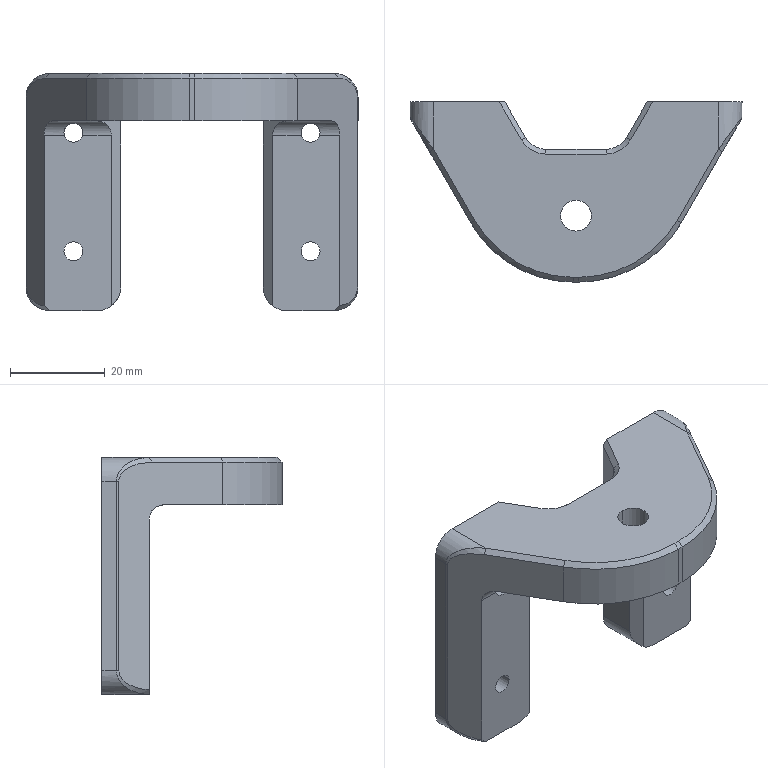Component | SolidWorks | DZ.KX.203-TC1505-30-09-01-05-28-2 | 1 solid | 68 faces | volume 29569 mm3 | plane 31 | cylinder 29 | spline 4 | cone 4 | commonest cylinder face diameters 4 x12 10 x8 16 x3 6.5 x2 50 x2 6 x2 | material Cast Carbon Steel